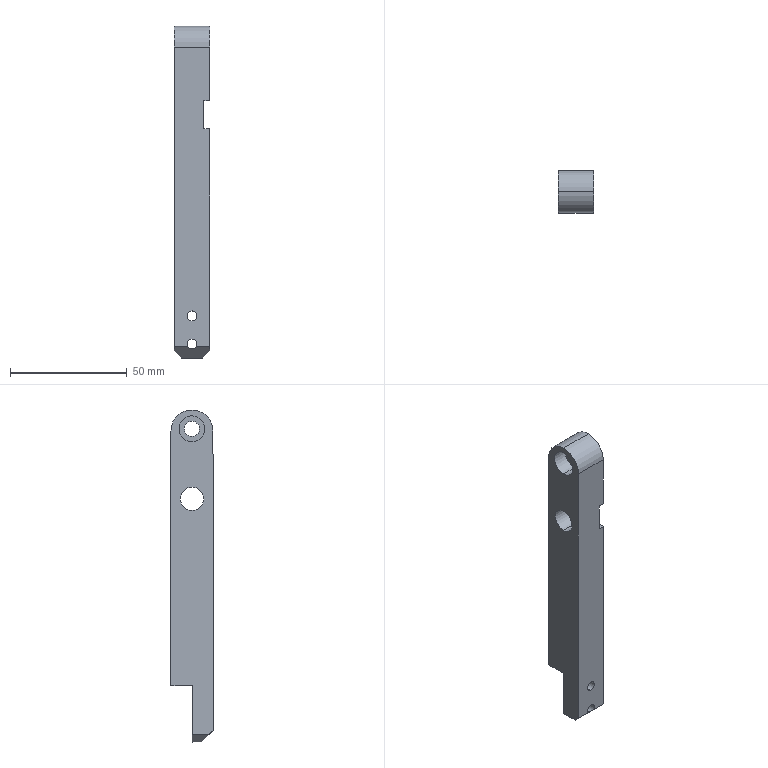Component | SolidWorks | ClampingArm2-1_A87-1 | 1 solid | 30 faces | box 15 x 18.04 x 142 mm | volume 31435 mm3 | plane 16 | cylinder 14 | commonest cylinder face diameters 4.2 x4 11 x2 14 x2 10 x2 6.5 x2 18 x2 | material S45C
STEP:
#1=COLOUR_RGB('',0.7922,0.8196,0.9333);
#2=FILL_AREA_STYLE_COLOUR('',#1);
#3=FILL_AREA_STYLE('',(#2));
#4=SURFACE_STYLE_FILL_AREA(#3);
#5=SURFACE_SIDE_STYLE('',(#4));
#6=SURFACE_STYLE_USAGE(.BOTH.,#5);
#7=PRESENTATION_STYLE_ASSIGNMENT((#6));
#8=CARTESIAN_POINT('',(-1.768,2.244,-5.964));
#9=VERTEX_POINT('',#8);
#10=CARTESIAN_POINT('',(-1.695,2.287,-6.008));
#11=VERTEX_POINT('',#10);
#12=CARTESIAN_POINT('',(-1.768,2.244,-5.964));
#13=CARTESIAN_POINT('',(-1.753,2.272,-5.992));
#14=CARTESIAN_POINT('',(-1.726,2.287,-6.008));
#15=CARTESIAN_POINT('',(-1.695,2.287,-6.008));
#16=(BOUNDED_CURVE()B_SPLINE_CURVE(3,(#12,#13,#14,#15),.UNSPECIFIED.,.F.,.F.)B_SPLINE_CURVE_WITH_KNOTS((4,4),(5.209,6.283),.UNSPECIFIED.)CURVE()GEOMETRIC_REPRESENTATION_ITEM()RATIONAL_B_SPLINE_CURVE((1.,0.9061,0.9061,1.))REPRESENTATION_ITEM(''));
#17=EDGE_CURVE('',#9,#11,#16,.T.);
#18=ORIENTED_EDGE('',*,*,#17,.T.);
#19=CARTESIAN_POINT('',(-1.695,2.599,-6.008));
#20=VERTEX_POINT('',#19);
#21=CARTESIAN_POINT('',(-1.695,2.599,-6.008));
#22=DIRECTION('',(-0.,1.,-0.0003333));
#23=VECTOR('',#22,39.37);
#24=LINE('',#21,#23);
#25=EDGE_CURVE('',#11,#20,#24,.T.);
#26=ORIENTED_EDGE('',*,*,#25,.T.);
#27=CARTESIAN_POINT('',(-1.695,2.599,-5.843));
#28=VERTEX_POINT('',#27);
#29=CARTESIAN_POINT('',(-1.695,2.599,-5.925));
#30=DIRECTION('',(-0.,1.,-0.0003333));
#31=DIRECTION('',(0.,0.0003333,1.));
#32=AXIS2_PLACEMENT_3D('',#29,#30,#31);
#33=CIRCLE('',#32,0.08268);
#34=EDGE_CURVE('',#20,#28,#33,.T.);
#35=ORIENTED_EDGE('',*,*,#34,.T.);
#36=CARTESIAN_POINT('',(-1.695,2.244,-5.842));
#37=VERTEX_POINT('',#36);
#38=CARTESIAN_POINT('',(-1.695,2.599,-5.843));
#39=DIRECTION('',(-0.,1.,-0.0003333));
#40=VECTOR('',#39,39.37);
#41=LINE('',#38,#40);
#42=EDGE_CURVE('',#37,#28,#41,.T.);
#43=ORIENTED_EDGE('',*,*,#42,.F.);
#44=CARTESIAN_POINT('',(-1.695,2.244,-5.925));
#45=DIRECTION('',(-0.,1.,-0.0003333));
#46=DIRECTION('',(0.,0.0003333,1.));
#47=AXIS2_PLACEMENT_3D('',#44,#45,#46);
#48=CIRCLE('',#47,0.08268);
#49=EDGE_CURVE('',#9,#37,#48,.T.);
#50=ORIENTED_EDGE('',*,*,#49,.F.);
#51=EDGE_LOOP('',(#18,#26,#35,#43,#50));
#52=FACE_OUTER_BOUND('',#51,.T.);
#53=CARTESIAN_POINT('',(-1.695,2.599,-5.925));
#54=DIRECTION('',(-0.,1.,-0.0003333));
#55=DIRECTION('',(0.,0.0003333,1.));
#56=AXIS2_PLACEMENT_3D('',#53,#54,#55);
#57=CYLINDRICAL_SURFACE('',#56,0.08268);
#58=ADVANCED_FACE('',(#52),#57,.F.);
#59=CARTESIAN_POINT('',(-1.695,2.244,-5.535));
#60=VERTEX_POINT('',#59);
#61=CARTESIAN_POINT('',(-1.695,2.244,-5.37));
#62=VERTEX_POINT('',#61);
#63=CARTESIAN_POINT('',(-1.695,2.244,-5.453));
#64=DIRECTION('',(-0.,1.,-0.0003333));
#65=DIRECTION('',(0.,0.0003333,1.));
#66=AXIS2_PLACEMENT_3D('',#63,#64,#65);
#67=CIRCLE('',#66,0.08268);
#68=EDGE_CURVE('',#60,#62,#67,.T.);
#69=ORIENTED_EDGE('',*,*,#68,.F.);
#70=CARTESIAN_POINT('',(-1.695,2.599,-5.535));
#71=VERTEX_POINT('',#70);
#72=CARTESIAN_POINT('',(-1.695,2.599,-5.535));
#73=DIRECTION('',(-0.,1.,-0.0003333));
#74=VECTOR('',#73,39.37);
#75=LINE('',#72,#74);
#76=EDGE_CURVE('',#60,#71,#75,.T.);
#77=ORIENTED_EDGE('',*,*,#76,.T.);
#78=CARTESIAN_POINT('',(-1.695,2.599,-5.37));
#79=VERTEX_POINT('',#78);
#80=CARTESIAN_POINT('',(-1.695,2.599,-5.453));
#81=DIRECTION('',(-0.,1.,-0.0003333));
#82=DIRECTION('',(0.,0.0003333,1.));
#83=AXIS2_PLACEMENT_3D('',#80,#81,#82);
#84=CIRCLE('',#83,0.08268);
#85=EDGE_CURVE('',#71,#79,#84,.T.);
#86=ORIENTED_EDGE('',*,*,#85,.T.);
#87=CARTESIAN_POINT('',(-1.695,2.599,-5.37));
#88=DIRECTION('',(-0.,1.,-0.0003333));
#89=VECTOR('',#88,39.37);
#90=LINE('',#87,#89);
#91=EDGE_CURVE('',#62,#79,#90,.T.);
#92=ORIENTED_EDGE('',*,*,#91,.F.);
#93=EDGE_LOOP('',(#69,#77,#86,#92));
#94=FACE_OUTER_BOUND('',#93,.T.);
#95=CARTESIAN_POINT('',(-1.695,2.599,-5.453));
#96=DIRECTION('',(-0.,1.,-0.0003333));
#97=DIRECTION('',(0.,0.0003333,1.));
#98=AXIS2_PLACEMENT_3D('',#95,#96,#97);
#99=CYLINDRICAL_SURFACE('',#98,0.08268);
#100=ADVANCED_FACE('',(#94),#99,.F.);
#101=CARTESIAN_POINT('',(-1.734,2.6,-1.102));
#102=VERTEX_POINT('',#101);
#103=CARTESIAN_POINT('',(-1.734,2.6,-0.6693));
#104=VERTEX_POINT('',#103);
#105=CARTESIAN_POINT('',(-1.734,2.6,-0.8858));
#106=DIRECTION('',(-1.,-0.,0.));
#107=DIRECTION('',(0.,0.0003333,1.));
#108=AXIS2_PLACEMENT_3D('',#105,#106,#107);
#109=CIRCLE('',#108,0.2165);
#110=EDGE_CURVE('',#102,#104,#109,.T.);
#111=ORIENTED_EDGE('',*,*,#110,.F.);
#112=CARTESIAN_POINT('',(-1.99,2.6,-1.102));
#113=VERTEX_POINT('',#112);
#114=CARTESIAN_POINT('',(-1.734,2.6,-1.102));
#115=DIRECTION('',(-1.,-0.,0.));
#116=VECTOR('',#115,39.37);
#117=LINE('',#114,#116);
#118=EDGE_CURVE('',#102,#113,#117,.T.);
#119=ORIENTED_EDGE('',*,*,#118,.T.);
#120=CARTESIAN_POINT('',(-1.99,2.6,-0.6693));
#121=VERTEX_POINT('',#120);
#122=CARTESIAN_POINT('',(-1.99,2.6,-0.8858));
#123=DIRECTION('',(-1.,-0.,0.));
#124=DIRECTION('',(0.,0.0003333,1.));
#125=AXIS2_PLACEMENT_3D('',#122,#123,#124);
#126=CIRCLE('',#125,0.2165);
#127=EDGE_CURVE('',#113,#121,#126,.T.);
#128=ORIENTED_EDGE('',*,*,#127,.T.);
#129=CARTESIAN_POINT('',(-1.734,2.6,-0.6693));
#130=DIRECTION('',(-1.,-0.,0.));
#131=VECTOR('',#130,39.37);
#132=LINE('',#129,#131);
#133=EDGE_CURVE('',#104,#121,#132,.T.);
#134=ORIENTED_EDGE('',*,*,#133,.F.);
#135=EDGE_LOOP('',(#111,#119,#128,#134));
#136=FACE_OUTER_BOUND('',#135,.T.);
#137=CARTESIAN_POINT('',(-1.734,2.6,-0.8858));
#138=DIRECTION('',(-1.,-0.,0.));
#139=DIRECTION('',(0.,0.0003333,1.));
#140=AXIS2_PLACEMENT_3D('',#137,#138,#139);
#141=CYLINDRICAL_SURFACE('',#140,0.2165);
#142=ADVANCED_FACE('',(#136),#141,.F.);
#143=CARTESIAN_POINT('',(-1.478,2.6,-0.6102));
#144=VERTEX_POINT('',#143);
#145=CARTESIAN_POINT('',(-1.478,2.6,-1.161));
#146=VERTEX_POINT('',#145);
#147=CARTESIAN_POINT('',(-1.478,2.6,-0.8858));
#148=DIRECTION('',(1.,0.,-0.));
#149=DIRECTION('',(0.,-0.0003333,-1.));
#150=AXIS2_PLACEMENT_3D('',#147,#148,#149);
#151=CIRCLE('',#150,0.2756);
#152=EDGE_CURVE('',#144,#146,#151,.T.);
#153=ORIENTED_EDGE('',*,*,#152,.F.);
#154=CARTESIAN_POINT('',(-1.4,2.6,-0.6102));
#155=VERTEX_POINT('',#154);
#156=CARTESIAN_POINT('',(-1.478,2.6,-0.6102));
#157=DIRECTION('',(1.,0.,-0.));
#158=VECTOR('',#157,39.37);
#159=LINE('',#156,#158);
#160=EDGE_CURVE('',#144,#155,#159,.T.);
#161=ORIENTED_EDGE('',*,*,#160,.T.);
#162=CARTESIAN_POINT('',(-1.4,2.6,-1.161));
#163=VERTEX_POINT('',#162);
#164=CARTESIAN_POINT('',(-1.4,2.6,-0.8858));
#165=DIRECTION('',(1.,0.,-0.));
#166=DIRECTION('',(0.,-0.0003333,-1.));
#167=AXIS2_PLACEMENT_3D('',#164,#165,#166);
#168=CIRCLE('',#167,0.2756);
#169=EDGE_CURVE('',#155,#163,#168,.T.);
#170=ORIENTED_EDGE('',*,*,#169,.T.);
#171=CARTESIAN_POINT('',(-1.478,2.6,-1.161));
#172=DIRECTION('',(1.,0.,-0.));
#173=VECTOR('',#172,39.37);
#174=LINE('',#171,#173);
#175=EDGE_CURVE('',#146,#163,#174,.T.);
#176=ORIENTED_EDGE('',*,*,#175,.F.);
#177=EDGE_LOOP('',(#153,#161,#170,#176));
#178=FACE_OUTER_BOUND('',#177,.T.);
#179=CARTESIAN_POINT('',(-1.478,2.6,-0.8858));
#180=DIRECTION('',(1.,0.,-0.));
#181=DIRECTION('',(0.,-0.0003333,-1.));
#182=AXIS2_PLACEMENT_3D('',#179,#180,#181);
#183=CYLINDRICAL_SURFACE('',#182,0.2756);
#184=ADVANCED_FACE('',(#178),#183,.F.);
#185=CARTESIAN_POINT('',(-1.99,2.6,-1.87));
#186=VERTEX_POINT('',#185);
#187=CARTESIAN_POINT('',(-1.99,2.6,-2.264));
#188=VERTEX_POINT('',#187);
#189=CARTESIAN_POINT('',(-1.99,2.6,-2.067));
#190=DIRECTION('',(1.,0.,-0.));
#191=DIRECTION('',(0.,-0.0003333,-1.));
#192=AXIS2_PLACEMENT_3D('',#189,#190,#191);
#193=CIRCLE('',#192,0.1969);
#194=EDGE_CURVE('',#186,#188,#193,.T.);
#195=ORIENTED_EDGE('',*,*,#194,.F.);
#196=CARTESIAN_POINT('',(-1.498,2.6,-1.87));
#197=VERTEX_POINT('',#196);
#198=CARTESIAN_POINT('',(-1.99,2.6,-1.87));
#199=DIRECTION('',(1.,0.,-0.));
#200=VECTOR('',#199,39.37);
#201=LINE('',#198,#200);
#202=EDGE_CURVE('',#186,#197,#201,.T.);
#203=ORIENTED_EDGE('',*,*,#202,.T.);
#204=CARTESIAN_POINT('',(-1.498,2.6,-2.264));
#205=VERTEX_POINT('',#204);
#206=CARTESIAN_POINT('',(-1.498,2.6,-2.067));
#207=DIRECTION('',(1.,0.,-0.));
#208=DIRECTION('',(0.,0.0003333,1.));
#209=AXIS2_PLACEMENT_3D('',#206,#207,#208);
#210=CIRCLE('',#209,0.1969);
#211=EDGE_CURVE('',#197,#205,#210,.T.);
#212=ORIENTED_EDGE('',*,*,#211,.T.);
#213=CARTESIAN_POINT('',(-1.99,2.6,-2.264));
#214=DIRECTION('',(1.,0.,-0.));
#215=VECTOR('',#214,39.37);
#216=LINE('',#213,#215);
#217=EDGE_CURVE('',#188,#205,#216,.T.);
#218=ORIENTED_EDGE('',*,*,#217,.F.);
#219=EDGE_LOOP('',(#195,#203,#212,#218));
#220=FACE_OUTER_BOUND('',#219,.T.);
#221=CARTESIAN_POINT('',(-1.99,2.6,-2.067));
#222=DIRECTION('',(1.,0.,-0.));
#223=DIRECTION('',(0.,-0.0003333,-1.));
#224=AXIS2_PLACEMENT_3D('',#221,#222,#223);
#225=CYLINDRICAL_SURFACE('',#224,0.1969);
#226=ADVANCED_FACE('',(#220),#225,.F.);
#227=CARTESIAN_POINT('',(-1.734,2.6,-0.7579));
#228=VERTEX_POINT('',#227);
#229=CARTESIAN_POINT('',(-1.734,2.6,-1.014));
#230=VERTEX_POINT('',#229);
#231=CARTESIAN_POINT('',(-1.734,2.6,-0.8858));
#232=DIRECTION('',(1.,0.,-0.));
#233=DIRECTION('',(0.,0.0003333,1.));
#234=AXIS2_PLACEMENT_3D('',#231,#232,#233);
#235=CIRCLE('',#234,0.128);
#236=EDGE_CURVE('',#228,#230,#235,.T.);
#237=ORIENTED_EDGE('',*,*,#236,.F.);
#238=CARTESIAN_POINT('',(-1.478,2.6,-0.7579));
#239=VERTEX_POINT('',#238);
#240=CARTESIAN_POINT('',(-1.99,2.6,-0.7579));
#241=DIRECTION('',(1.,0.,-0.));
#242=VECTOR('',#241,39.37);
#243=LINE('',#240,#242);
#244=EDGE_CURVE('',#228,#239,#243,.T.);
#245=ORIENTED_EDGE('',*,*,#244,.T.);
#246=CARTESIAN_POINT('',(-1.478,2.6,-1.014));
#247=VERTEX_POINT('',#246);
#248=CARTESIAN_POINT('',(-1.478,2.6,-0.8858));
#249=DIRECTION('',(-1.,-0.,0.));
#250=DIRECTION('',(0.,-0.0003333,-1.));
#251=AXIS2_PLACEMENT_3D('',#248,#249,#250);
#252=CIRCLE('',#251,0.128);
#253=EDGE_CURVE('',#247,#239,#252,.T.);
#254=ORIENTED_EDGE('',*,*,#253,.F.);
#255=CARTESIAN_POINT('',(-1.99,2.6,-1.014));
#256=DIRECTION('',(1.,0.,-0.));
#257=VECTOR('',#256,39.37);
#258=LINE('',#255,#257);
#259=EDGE_CURVE('',#230,#247,#258,.T.);
#260=ORIENTED_EDGE('',*,*,#259,.F.);
#261=EDGE_LOOP('',(#237,#245,#254,#260));
#262=FACE_OUTER_BOUND('',#261,.T.);
#263=CARTESIAN_POINT('',(-1.99,2.6,-0.8858));
#264=DIRECTION('',(1.,0.,-0.));
#265=DIRECTION('',(0.,-0.0003333,-1.));
#266=AXIS2_PLACEMENT_3D('',#263,#264,#265);
#267=CYLINDRICAL_SURFACE('',#266,0.128);
#268=ADVANCED_FACE('',(#262),#267,.F.);
#269=ORIENTED_EDGE('',*,*,#244,.F.);
#270=CARTESIAN_POINT('',(-1.734,2.6,-0.8858));
#271=DIRECTION('',(1.,0.,-0.));
#272=DIRECTION('',(0.,0.0003333,1.));
#273=AXIS2_PLACEMENT_3D('',#270,#271,#272);
#274=CIRCLE('',#273,0.128);
#275=EDGE_CURVE('',#230,#228,#274,.T.);
#276=ORIENTED_EDGE('',*,*,#275,.F.);
#277=ORIENTED_EDGE('',*,*,#259,.T.);
#278=CARTESIAN_POINT('',(-1.478,2.6,-0.8858));
#279=DIRECTION('',(-1.,-0.,0.));
#280=DIRECTION('',(0.,-0.0003333,-1.));
#281=AXIS2_PLACEMENT_3D('',#278,#279,#280);
#282=CIRCLE('',#281,0.128);
#283=EDGE_CURVE('',#239,#247,#282,.T.);
#284=ORIENTED_EDGE('',*,*,#283,.F.);
#285=EDGE_LOOP('',(#269,#276,#277,#284));
#286=FACE_OUTER_BOUND('',#285,.T.);
#287=CARTESIAN_POINT('',(-1.99,2.6,-0.8858));
#288=DIRECTION('',(1.,0.,-0.));
#289=DIRECTION('',(0.,-0.0003333,-1.));
#290=AXIS2_PLACEMENT_3D('',#287,#288,#289);
#291=CYLINDRICAL_SURFACE('',#290,0.128);
#292=ADVANCED_FACE('',(#286),#291,.F.);
#293=CARTESIAN_POINT('',(-1.4,2.6,-0.8858));
#294=DIRECTION('',(1.,0.,-0.));
#295=DIRECTION('',(0.,-0.0003333,-1.));
#296=AXIS2_PLACEMENT_3D('',#293,#294,#295);
#297=CIRCLE('',#296,0.2756);
#298=EDGE_CURVE('',#163,#155,#297,.T.);
#299=ORIENTED_EDGE('',*,*,#298,.F.);
#300=ORIENTED_EDGE('',*,*,#169,.F.);
#301=EDGE_LOOP('',(#299,#300));
#302=FACE_BOUND('',#301,.T.);
#303=CARTESIAN_POINT('',(-1.4,2.954,-1.831));
#304=VERTEX_POINT('',#303);
#305=CARTESIAN_POINT('',(-1.4,2.955,-0.9253));
#306=VERTEX_POINT('',#305);
#307=CARTESIAN_POINT('',(-1.4,2.955,-0.571));
#308=DIRECTION('',(0.,0.0003333,1.));
#309=VECTOR('',#308,39.37);
#310=LINE('',#307,#309);
#311=EDGE_CURVE('',#304,#306,#310,.T.);
#312=ORIENTED_EDGE('',*,*,#311,.T.);
#313=CARTESIAN_POINT('',(-1.4,2.6,-0.5709));
#314=VERTEX_POINT('',#313);
#315=CARTESIAN_POINT('',(-1.4,2.6,-0.9252));
#316=DIRECTION('',(1.,0.,-0.));
#317=DIRECTION('',(0.,-0.0003333,-1.));
#318=AXIS2_PLACEMENT_3D('',#315,#316,#317);
#319=CIRCLE('',#318,0.3543);
#320=EDGE_CURVE('',#306,#314,#319,.T.);
#321=ORIENTED_EDGE('',*,*,#320,.T.);
#322=CARTESIAN_POINT('',(-1.4,2.246,-0.9251));
#323=VERTEX_POINT('',#322);
#324=CARTESIAN_POINT('',(-1.4,2.6,-0.9252));
#325=DIRECTION('',(1.,0.,-0.));
#326=DIRECTION('',(0.,-0.0003333,-1.));
#327=AXIS2_PLACEMENT_3D('',#324,#325,#326);
#328=CIRCLE('',#327,0.3543);
#329=EDGE_CURVE('',#314,#323,#328,.T.);
#330=ORIENTED_EDGE('',*,*,#329,.T.);
#331=CARTESIAN_POINT('',(-1.4,2.246,-1.831));
#332=VERTEX_POINT('',#331);
#333=CARTESIAN_POINT('',(-1.4,2.246,-0.5707));
#334=DIRECTION('',(-0.,-0.0003333,-1.));
#335=VECTOR('',#334,39.37);
#336=LINE('',#333,#335);
#337=EDGE_CURVE('',#323,#332,#336,.T.);
#338=ORIENTED_EDGE('',*,*,#337,.T.);
#339=CARTESIAN_POINT('',(-1.4,2.954,-1.831));
#340=DIRECTION('',(0.,-1.,0.0003333));
#341=VECTOR('',#340,39.37);
#342=LINE('',#339,#341);
#343=EDGE_CURVE('',#304,#332,#342,.T.);
#344=ORIENTED_EDGE('',*,*,#343,.F.);
#345=EDGE_LOOP('',(#312,#321,#330,#338,#344));
#346=FACE_OUTER_BOUND('',#345,.T.);
#347=CARTESIAN_POINT('',(-1.4,2.599,-3.366));
#348=DIRECTION('',(1.,0.,-0.));
#349=DIRECTION('',(-0.,-0.0003333,-1.));
#350=AXIS2_PLACEMENT_3D('',#347,#348,#349);
#351=PLANE('',#350);
#352=ADVANCED_FACE('',(#302,#346),#351,.T.);
#353=CARTESIAN_POINT('',(-1.518,2.598,-6.161));
#354=VERTEX_POINT('',#353);
#355=CARTESIAN_POINT('',(-1.518,2.441,-6.161));
#356=VERTEX_POINT('',#355);
#357=CARTESIAN_POINT('',(-1.518,2.244,-6.161));
#358=DIRECTION('',(0.,-1.,0.0003333));
#359=VECTOR('',#358,39.37);
#360=LINE('',#357,#359);
#361=EDGE_CURVE('',#354,#356,#360,.T.);
#362=ORIENTED_EDGE('',*,*,#361,.T.);
#363=CARTESIAN_POINT('',(-1.872,2.441,-6.161));
#364=VERTEX_POINT('',#363);
#365=CARTESIAN_POINT('',(-1.4,2.441,-6.161));
#366=DIRECTION('',(-1.,-0.,0.));
#367=VECTOR('',#366,39.37);
#368=LINE('',#365,#367);
#369=EDGE_CURVE('',#356,#364,#368,.T.);
#370=ORIENTED_EDGE('',*,*,#369,.T.);
#371=CARTESIAN_POINT('',(-1.872,2.598,-6.161));
#372=VERTEX_POINT('',#371);
#373=CARTESIAN_POINT('',(-1.872,2.953,-6.162));
#374=DIRECTION('',(-0.,1.,-0.0003333));
#375=VECTOR('',#374,39.37);
#376=LINE('',#373,#375);
#377=EDGE_CURVE('',#364,#372,#376,.T.);
#378=ORIENTED_EDGE('',*,*,#377,.T.);
#379=CARTESIAN_POINT('',(-1.99,2.598,-6.161));
#380=DIRECTION('',(1.,0.,-0.));
#381=VECTOR('',#380,39.37);
#382=LINE('',#379,#381);
#383=EDGE_CURVE('',#372,#354,#382,.T.);
#384=ORIENTED_EDGE('',*,*,#383,.T.);
#385=EDGE_LOOP('',(#362,#370,#378,#384));
#386=FACE_OUTER_BOUND('',#385,.T.);
#387=CARTESIAN_POINT('',(-1.4,2.953,-6.162));
#388=DIRECTION('',(0.,0.0003333,1.));
#389=DIRECTION('',(1.,0.,-0.));
#390=AXIS2_PLACEMENT_3D('',#387,#388,#389);
#391=PLANE('',#390);
#392=ADVANCED_FACE('',(#386),#391,.F.);
#393=CARTESIAN_POINT('',(-1.4,2.953,-5.217));
#394=VERTEX_POINT('',#393);
#395=CARTESIAN_POINT('',(-1.4,2.954,-2.303));
#396=VERTEX_POINT('',#395);
#397=CARTESIAN_POINT('',(-1.4,2.955,-0.571));
#398=DIRECTION('',(0.,0.0003333,1.));
#399=VECTOR('',#398,39.37);
#400=LINE('',#397,#399);
#401=EDGE_CURVE('',#394,#396,#400,.T.);
#402=ORIENTED_EDGE('',*,*,#401,.F.);
#403=CARTESIAN_POINT('',(-1.99,2.953,-5.217));
#404=VERTEX_POINT('',#403);
#405=CARTESIAN_POINT('',(-1.99,2.953,-5.217));
#406=DIRECTION('',(1.,0.,-0.));
#407=VECTOR('',#406,39.37);
#408=LINE('',#405,#407);
#409=EDGE_CURVE('',#404,#394,#408,.T.);
#410=ORIENTED_EDGE('',*,*,#409,.F.);
#411=CARTESIAN_POINT('',(-1.99,2.955,-0.9253));
#412=VERTEX_POINT('',#411);
#413=CARTESIAN_POINT('',(-1.99,2.955,-0.571));
#414=DIRECTION('',(0.,0.0003333,1.));
#415=VECTOR('',#414,39.37);
#416=LINE('',#413,#415);
#417=EDGE_CURVE('',#404,#412,#416,.T.);
#418=ORIENTED_EDGE('',*,*,#417,.T.);
#419=CARTESIAN_POINT('',(-1.4,2.955,-0.9253));
#420=DIRECTION('',(1.,0.,-0.));
#421=VECTOR('',#420,39.37);
#422=LINE('',#419,#421);
#423=EDGE_CURVE('',#412,#306,#422,.T.);
#424=ORIENTED_EDGE('',*,*,#423,.T.);
#425=ORIENTED_EDGE('',*,*,#311,.F.);
#426=CARTESIAN_POINT('',(-1.498,2.954,-1.831));
#427=VERTEX_POINT('',#426);
#428=CARTESIAN_POINT('',(-1.498,2.954,-1.831));
#429=DIRECTION('',(1.,0.,-0.));
#430=VECTOR('',#429,39.37);
#431=LINE('',#428,#430);
#432=EDGE_CURVE('',#427,#304,#431,.T.);
#433=ORIENTED_EDGE('',*,*,#432,.F.);
#434=CARTESIAN_POINT('',(-1.498,2.954,-2.303));
#435=VERTEX_POINT('',#434);
#436=CARTESIAN_POINT('',(-1.498,2.954,-2.303));
#437=DIRECTION('',(0.,0.0003333,1.));
#438=VECTOR('',#437,39.37);
#439=LINE('',#436,#438);
#440=EDGE_CURVE('',#435,#427,#439,.T.);
#441=ORIENTED_EDGE('',*,*,#440,.F.);
#442=CARTESIAN_POINT('',(-1.498,2.954,-2.303));
#443=DIRECTION('',(1.,0.,-0.));
#444=VECTOR('',#443,39.37);
#445=LINE('',#442,#444);
#446=EDGE_CURVE('',#435,#396,#445,.T.);
#447=ORIENTED_EDGE('',*,*,#446,.T.);
#448=EDGE_LOOP('',(#402,#410,#418,#424,#425,#433,#441,#447));
#449=FACE_OUTER_BOUND('',#448,.T.);
#450=CARTESIAN_POINT('',(-1.4,2.955,-0.571));
#451=DIRECTION('',(0.,-1.,0.0003333));
#452=DIRECTION('',(-0.,-0.0003333,-1.));
#453=AXIS2_PLACEMENT_3D('',#450,#451,#452);
#454=PLANE('',#453);
#455=ADVANCED_FACE('',(#449),#454,.F.);
#456=CARTESIAN_POINT('',(-1.695,2.244,-5.453));
#457=DIRECTION('',(-0.,1.,-0.0003333));
#458=DIRECTION('',(0.,0.0003333,1.));
#459=AXIS2_PLACEMENT_3D('',#456,#457,#458);
#460=CIRCLE('',#459,0.08268);
#461=EDGE_CURVE('',#62,#60,#460,.T.);
#462=ORIENTED_EDGE('',*,*,#461,.T.);
#463=ORIENTED_EDGE('',*,*,#68,.T.);
#464=EDGE_LOOP('',(#462,#463));
#465=FACE_BOUND('',#464,.T.);
#466=CARTESIAN_POINT('',(-1.99,2.244,-5.964));
#467=VERTEX_POINT('',#466);
#468=CARTESIAN_POINT('',(-1.4,2.244,-5.964));
#469=DIRECTION('',(1.,0.,-0.));
#470=VECTOR('',#469,39.37);
#471=LINE('',#468,#470);
#472=EDGE_CURVE('',#467,#9,#471,.T.);
#473=ORIENTED_EDGE('',*,*,#472,.T.);
#474=ORIENTED_EDGE('',*,*,#49,.T.);
#475=CARTESIAN_POINT('',(-1.622,2.244,-5.964));
#476=VERTEX_POINT('',#475);
#477=CARTESIAN_POINT('',(-1.695,2.244,-5.925));
#478=DIRECTION('',(-0.,1.,-0.0003333));
#479=DIRECTION('',(0.,0.0003333,1.));
#480=AXIS2_PLACEMENT_3D('',#477,#478,#479);
#481=CIRCLE('',#480,0.08268);
#482=EDGE_CURVE('',#37,#476,#481,.T.);
#483=ORIENTED_EDGE('',*,*,#482,.T.);
#484=CARTESIAN_POINT('',(-1.4,2.244,-5.964));
#485=VERTEX_POINT('',#484);
#486=CARTESIAN_POINT('',(-1.4,2.244,-5.964));
#487=DIRECTION('',(1.,0.,-0.));
#488=VECTOR('',#487,39.37);
#489=LINE('',#486,#488);
#490=EDGE_CURVE('',#476,#485,#489,.T.);
#491=ORIENTED_EDGE('',*,*,#490,.T.);
#492=CARTESIAN_POINT('',(-1.4,2.245,-2.303));
#493=VERTEX_POINT('',#492);
#494=CARTESIAN_POINT('',(-1.4,2.246,-0.5707));
#495=DIRECTION('',(-0.,-0.0003333,-1.));
#496=VECTOR('',#495,39.37);
#497=LINE('',#494,#496);
#498=EDGE_CURVE('',#493,#485,#497,.T.);
#499=ORIENTED_EDGE('',*,*,#498,.F.);
#500=CARTESIAN_POINT('',(-1.498,2.245,-2.303));
#501=VERTEX_POINT('',#500);
#502=CARTESIAN_POINT('',(-1.498,2.245,-2.303));
#503=DIRECTION('',(1.,0.,-0.));
#504=VECTOR('',#503,39.37);
#505=LINE('',#502,#504);
#506=EDGE_CURVE('',#501,#493,#505,.T.);
#507=ORIENTED_EDGE('',*,*,#506,.F.);
#508=CARTESIAN_POINT('',(-1.498,2.246,-1.831));
#509=VERTEX_POINT('',#508);
#510=CARTESIAN_POINT('',(-1.498,2.245,-2.303));
#511=DIRECTION('',(-0.,-0.0003333,-1.));
#512=VECTOR('',#511,39.37);
#513=LINE('',#510,#512);
#514=EDGE_CURVE('',#509,#501,#513,.T.);
#515=ORIENTED_EDGE('',*,*,#514,.F.);
#516=CARTESIAN_POINT('',(-1.498,2.246,-1.831));
#517=DIRECTION('',(1.,0.,-0.));
#518=VECTOR('',#517,39.37);
#519=LINE('',#516,#518);
#520=EDGE_CURVE('',#509,#332,#519,.T.);
#521=ORIENTED_EDGE('',*,*,#520,.T.);
#522=ORIENTED_EDGE('',*,*,#337,.F.);
#523=CARTESIAN_POINT('',(-1.99,2.246,-0.9251));
#524=VERTEX_POINT('',#523);
#525=CARTESIAN_POINT('',(-1.4,2.246,-0.9251));
#526=DIRECTION('',(-1.,-0.,0.));
#527=VECTOR('',#526,39.37);
#528=LINE('',#525,#527);
#529=EDGE_CURVE('',#323,#524,#528,.T.);
#530=ORIENTED_EDGE('',*,*,#529,.T.);
#531=CARTESIAN_POINT('',(-1.99,2.246,-0.5707));
#532=DIRECTION('',(-0.,-0.0003333,-1.));
#533=VECTOR('',#532,39.37);
#534=LINE('',#531,#533);
#535=EDGE_CURVE('',#524,#467,#534,.T.);
#536=ORIENTED_EDGE('',*,*,#535,.T.);
#537=EDGE_LOOP('',(#473,#474,#483,#491,#499,#507,#515,#521,#522,#530,#536));
#538=FACE_OUTER_BOUND('',#537,.T.);
#539=CARTESIAN_POINT('',(-1.4,2.246,-0.5707));
#540=DIRECTION('',(-0.,1.,-0.0003333));
#541=DIRECTION('',(0.,0.0003333,1.));
#542=AXIS2_PLACEMENT_3D('',#539,#540,#541);
#543=PLANE('',#542);
#544=ADVANCED_FACE('',(#465,#538),#543,.F.);
#545=ORIENTED_EDGE('',*,*,#498,.T.);
#546=CARTESIAN_POINT('',(-1.4,2.323,-6.043));
#547=VERTEX_POINT('',#546);
#548=CARTESIAN_POINT('',(-1.4,1.123,-4.842));
#549=DIRECTION('',(-0.,0.7069,-0.7073));
#550=VECTOR('',#549,39.37);
#551=LINE('',#548,#550);
#552=EDGE_CURVE('',#485,#547,#551,.T.);
#553=ORIENTED_EDGE('',*,*,#552,.T.);
#554=CARTESIAN_POINT('',(-1.4,2.599,-6.043));
#555=VERTEX_POINT('',#554);
#556=CARTESIAN_POINT('',(-1.4,2.599,-6.043));
#557=DIRECTION('',(-0.,1.,-0.0003333));
#558=VECTOR('',#557,39.37);
#559=LINE('',#556,#558);
#560=EDGE_CURVE('',#547,#555,#559,.T.);
#561=ORIENTED_EDGE('',*,*,#560,.T.);
#562=CARTESIAN_POINT('',(-1.4,2.599,-5.217));
#563=VERTEX_POINT('',#562);
#564=CARTESIAN_POINT('',(-1.4,2.598,-6.161));
#565=DIRECTION('',(-0.,-0.0003333,-1.));
#566=VECTOR('',#565,39.37);
#567=LINE('',#564,#566);
#568=EDGE_CURVE('',#563,#555,#567,.T.);
#569=ORIENTED_EDGE('',*,*,#568,.F.);
#570=CARTESIAN_POINT('',(-1.4,2.953,-5.217));
#571=DIRECTION('',(0.,-1.,0.0003333));
#572=VECTOR('',#571,39.37);
#573=LINE('',#570,#572);
#574=EDGE_CURVE('',#394,#563,#573,.T.);
#575=ORIENTED_EDGE('',*,*,#574,.F.);
#576=ORIENTED_EDGE('',*,*,#401,.T.);
#577=CARTESIAN_POINT('',(-1.4,2.954,-2.303));
#578=DIRECTION('',(-0.,1.,-0.0003333));
#579=VECTOR('',#578,39.37);
#580=LINE('',#577,#579);
#581=EDGE_CURVE('',#493,#396,#580,.T.);
#582=ORIENTED_EDGE('',*,*,#581,.F.);
#583=EDGE_LOOP('',(#545,#553,#561,#569,#575,#576,#582));
#584=FACE_OUTER_BOUND('',#583,.T.);
#585=CARTESIAN_POINT('',(-1.4,2.599,-3.366));
#586=DIRECTION('',(1.,0.,-0.));
#587=DIRECTION('',(-0.,-0.0003333,-1.));
#588=AXIS2_PLACEMENT_3D('',#585,#586,#587);
#589=PLANE('',#588);
#590=ADVANCED_FACE('',(#584),#589,.T.);
#591=CARTESIAN_POINT('',(-1.99,2.6,-0.8858));
#592=DIRECTION('',(-1.,-0.,0.));
#593=DIRECTION('',(0.,0.0003333,1.));
#594=AXIS2_PLACEMENT_3D('',#591,#592,#593);
#595=CIRCLE('',#594,0.2165);
#596=EDGE_CURVE('',#121,#113,#595,.T.);
#597=ORIENTED_EDGE('',*,*,#596,.F.);
#598=ORIENTED_EDGE('',*,*,#127,.F.);
#599=EDGE_LOOP('',(#597,#598));
#600=FACE_BOUND('',#599,.T.);
#601=CARTESIAN_POINT('',(-1.99,2.6,-2.067));
#602=DIRECTION('',(1.,0.,-0.));
#603=DIRECTION('',(0.,-0.0003333,-1.));
#604=AXIS2_PLACEMENT_3D('',#601,#602,#603);
#605=CIRCLE('',#604,0.1969);
#606=EDGE_CURVE('',#188,#186,#605,.T.);
#607=ORIENTED_EDGE('',*,*,#606,.T.);
#608=ORIENTED_EDGE('',*,*,#194,.T.);
#609=EDGE_LOOP('',(#607,#608));
#610=FACE_BOUND('',#609,.T.);
#611=CARTESIAN_POINT('',(-1.99,2.599,-6.043));
#612=VERTEX_POINT('',#611);
#613=CARTESIAN_POINT('',(-1.99,2.323,-6.043));
#614=VERTEX_POINT('',#613);
#615=CARTESIAN_POINT('',(-1.99,2.599,-6.043));
#616=DIRECTION('',(0.,-1.,0.0003333));
#617=VECTOR('',#616,39.37);
#618=LINE('',#615,#617);
#619=EDGE_CURVE('',#612,#614,#618,.T.);
#620=ORIENTED_EDGE('',*,*,#619,.T.);
#621=CARTESIAN_POINT('',(-1.99,2.441,-6.161));
#622=DIRECTION('',(0.,-0.7069,0.7073));
#623=VECTOR('',#622,39.37);
#624=LINE('',#621,#623);
#625=EDGE_CURVE('',#614,#467,#624,.T.);
#626=ORIENTED_EDGE('',*,*,#625,.T.);
#627=ORIENTED_EDGE('',*,*,#535,.F.);
#628=CARTESIAN_POINT('',(-1.99,2.6,-0.5709));
#629=VERTEX_POINT('',#628);
#630=CARTESIAN_POINT('',(-1.99,2.6,-0.9252));
#631=DIRECTION('',(-1.,-0.,0.));
#632=DIRECTION('',(0.,-0.0003333,-1.));
#633=AXIS2_PLACEMENT_3D('',#630,#631,#632);
#634=CIRCLE('',#633,0.3543);
#635=EDGE_CURVE('',#524,#629,#634,.T.);
#636=ORIENTED_EDGE('',*,*,#635,.T.);
#637=CARTESIAN_POINT('',(-1.99,2.6,-0.9252));
#638=DIRECTION('',(-1.,-0.,0.));
#639=DIRECTION('',(0.,-0.0003333,-1.));
#640=AXIS2_PLACEMENT_3D('',#637,#638,#639);
#641=CIRCLE('',#640,0.3543);
#642=EDGE_CURVE('',#629,#412,#641,.T.);
#643=ORIENTED_EDGE('',*,*,#642,.T.);
#644=ORIENTED_EDGE('',*,*,#417,.F.);
#645=CARTESIAN_POINT('',(-1.99,2.599,-5.217));
#646=VERTEX_POINT('',#645);
#647=CARTESIAN_POINT('',(-1.99,2.953,-5.217));
#648=DIRECTION('',(0.,-1.,0.0003333));
#649=VECTOR('',#648,39.37);
#650=LINE('',#647,#649);
#651=EDGE_CURVE('',#404,#646,#650,.T.);
#652=ORIENTED_EDGE('',*,*,#651,.T.);
#653=CARTESIAN_POINT('',(-1.99,2.598,-6.161));
#654=DIRECTION('',(-0.,-0.0003333,-1.));
#655=VECTOR('',#654,39.37);
#656=LINE('',#653,#655);
#657=EDGE_CURVE('',#646,#612,#656,.T.);
#658=ORIENTED_EDGE('',*,*,#657,.T.);
#659=EDGE_LOOP('',(#620,#626,#627,#636,#643,#644,#652,#658));
#660=FACE_OUTER_BOUND('',#659,.T.);
#661=CARTESIAN_POINT('',(-1.99,2.599,-3.366));
#662=DIRECTION('',(1.,0.,-0.));
#663=DIRECTION('',(-0.,-0.0003333,-1.));
#664=AXIS2_PLACEMENT_3D('',#661,#662,#663);
#665=PLANE('',#664);
#666=ADVANCED_FACE('',(#600,#610,#660),#665,.F.);
#667=ORIENTED_EDGE('',*,*,#202,.F.);
#668=ORIENTED_EDGE('',*,*,#606,.F.);
#669=ORIENTED_EDGE('',*,*,#217,.T.);
#670=CARTESIAN_POINT('',(-1.498,2.6,-2.067));
#671=DIRECTION('',(1.,0.,-0.));
#672=DIRECTION('',(0.,0.0003333,1.));
#673=AXIS2_PLACEMENT_3D('',#670,#671,#672);
#674=CIRCLE('',#673,0.1969);
#675=EDGE_CURVE('',#205,#197,#674,.T.);
#676=ORIENTED_EDGE('',*,*,#675,.T.);
#677=EDGE_LOOP('',(#667,#668,#669,#676));
#678=FACE_OUTER_BOUND('',#677,.T.);
#679=CARTESIAN_POINT('',(-1.99,2.6,-2.067));
#680=DIRECTION('',(1.,0.,-0.));
#681=DIRECTION('',(0.,-0.0003333,-1.));
#682=AXIS2_PLACEMENT_3D('',#679,#680,#681);
#683=CYLINDRICAL_SURFACE('',#682,0.1969);
#684=ADVANCED_FACE('',(#678),#683,.F.);
#685=CARTESIAN_POINT('',(-1.498,2.954,-1.831));
#686=DIRECTION('',(0.,-1.,0.0003333));
#687=VECTOR('',#686,39.37);
#688=LINE('',#685,#687);
#689=EDGE_CURVE('',#427,#509,#688,.T.);
#690=ORIENTED_EDGE('',*,*,#689,.T.);
#691=ORIENTED_EDGE('',*,*,#514,.T.);
#692=CARTESIAN_POINT('',(-1.498,2.954,-2.303));
#693=DIRECTION('',(-0.,1.,-0.0003333));
#694=VECTOR('',#693,39.37);
#695=LINE('',#692,#694);
#696=EDGE_CURVE('',#501,#435,#695,.T.);
#697=ORIENTED_EDGE('',*,*,#696,.T.);
#698=ORIENTED_EDGE('',*,*,#440,.T.);
#699=EDGE_LOOP('',(#690,#691,#697,#698));
#700=FACE_OUTER_BOUND('',#699,.T.);
#701=ORIENTED_EDGE('',*,*,#675,.F.);
#702=ORIENTED_EDGE('',*,*,#211,.F.);
#703=EDGE_LOOP('',(#701,#702));
#704=FACE_BOUND('',#703,.T.);
#705=CARTESIAN_POINT('',(-1.498,2.599,-3.366));
#706=DIRECTION('',(-1.,-0.,0.));
#707=DIRECTION('',(0.,0.0003333,1.));
#708=AXIS2_PLACEMENT_3D('',#705,#706,#707);
#709=PLANE('',#708);
#710=ADVANCED_FACE('',(#700,#704),#709,.F.);
#711=ORIENTED_EDGE('',*,*,#343,.T.);
#712=ORIENTED_EDGE('',*,*,#520,.F.);
#713=ORIENTED_EDGE('',*,*,#689,.F.);
#714=ORIENTED_EDGE('',*,*,#432,.T.);
#715=EDGE_LOOP('',(#711,#712,#713,#714));
#716=FACE_OUTER_BOUND('',#715,.T.);
#717=CARTESIAN_POINT('',(-1.498,2.954,-1.831));
#718=DIRECTION('',(0.,0.0003333,1.));
#719=DIRECTION('',(1.,0.,-0.));
#720=AXIS2_PLACEMENT_3D('',#717,#718,#719);
#721=PLANE('',#720);
#722=ADVANCED_FACE('',(#716),#721,.F.);
#723=ORIENTED_EDGE('',*,*,#581,.T.);
#724=ORIENTED_EDGE('',*,*,#446,.F.);
#725=ORIENTED_EDGE('',*,*,#696,.F.);
#726=ORIENTED_EDGE('',*,*,#506,.T.);
#727=EDGE_LOOP('',(#723,#724,#725,#726));
#728=FACE_OUTER_BOUND('',#727,.T.);
#729=CARTESIAN_POINT('',(-1.498,2.954,-2.303));
#730=DIRECTION('',(-0.,-0.0003333,-1.));
#731=DIRECTION('',(-1.,-0.,0.));
#732=AXIS2_PLACEMENT_3D('',#729,#730,#731);
#733=PLANE('',#732);
#734=ADVANCED_FACE('',(#728),#733,.F.);
#735=ORIENTED_EDGE('',*,*,#529,.F.);
#736=ORIENTED_EDGE('',*,*,#329,.F.);
#737=CARTESIAN_POINT('',(-1.4,2.6,-0.5709));
#738=DIRECTION('',(1.,0.,-0.));
#739=VECTOR('',#738,39.37);
#740=LINE('',#737,#739);
#741=EDGE_CURVE('',#629,#314,#740,.T.);
#742=ORIENTED_EDGE('',*,*,#741,.F.);
#743=ORIENTED_EDGE('',*,*,#635,.F.);
#744=EDGE_LOOP('',(#735,#736,#742,#743));
#745=FACE_OUTER_BOUND('',#744,.T.);
#746=CARTESIAN_POINT('',(-1.4,2.6,-0.9252));
#747=DIRECTION('',(-1.,-0.,0.));
#748=DIRECTION('',(0.,0.0003333,1.));
#749=AXIS2_PLACEMENT_3D('',#746,#747,#748);
#750=CYLINDRICAL_SURFACE('',#749,0.3543);
#751=ADVANCED_FACE('',(#745),#750,.T.);
#752=ORIENTED_EDGE('',*,*,#320,.F.);
#753=ORIENTED_EDGE('',*,*,#423,.F.);
#754=ORIENTED_EDGE('',*,*,#642,.F.);
#755=ORIENTED_EDGE('',*,*,#741,.T.);
#756=EDGE_LOOP('',(#752,#753,#754,#755));
#757=FACE_OUTER_BOUND('',#756,.T.);
#758=CARTESIAN_POINT('',(-1.4,2.6,-0.9252));
#759=DIRECTION('',(-1.,-0.,0.));
#760=DIRECTION('',(0.,0.0003333,1.));
#761=AXIS2_PLACEMENT_3D('',#758,#759,#760);
#762=CYLINDRICAL_SURFACE('',#761,0.3543);
#763=ADVANCED_FACE('',(#757),#762,.T.);
#764=CARTESIAN_POINT('',(-1.478,2.6,-0.8858));
#765=DIRECTION('',(1.,0.,-0.));
#766=DIRECTION('',(0.,-0.0003333,-1.));
#767=AXIS2_PLACEMENT_3D('',#764,#765,#766);
#768=CIRCLE('',#767,0.2756);
#769=EDGE_CURVE('',#146,#144,#768,.T.);
#770=ORIENTED_EDGE('',*,*,#769,.T.);
#771=ORIENTED_EDGE('',*,*,#152,.T.);
#772=EDGE_LOOP('',(#770,#771));
#773=FACE_OUTER_BOUND('',#772,.T.);
#774=ORIENTED_EDGE('',*,*,#253,.T.);
#775=ORIENTED_EDGE('',*,*,#283,.T.);
#776=EDGE_LOOP('',(#774,#775));
#777=FACE_BOUND('',#776,.T.);
#778=CARTESIAN_POINT('',(-1.478,2.6,-0.8858));
#779=DIRECTION('',(1.,0.,-0.));
#780=DIRECTION('',(-0.,-0.0003333,-1.));
#781=AXIS2_PLACEMENT_3D('',#778,#779,#780);
#782=PLANE('',#781);
#783=ADVANCED_FACE('',(#773,#777),#782,.T.);
#784=ORIENTED_EDGE('',*,*,#160,.F.);
#785=ORIENTED_EDGE('',*,*,#769,.F.);
#786=ORIENTED_EDGE('',*,*,#175,.T.);
#787=ORIENTED_EDGE('',*,*,#298,.T.);
#788=EDGE_LOOP('',(#784,#785,#786,#787));
#789=FACE_OUTER_BOUND('',#788,.T.);
#790=CARTESIAN_POINT('',(-1.478,2.6,-0.8858));
#791=DIRECTION('',(1.,0.,-0.));
#792=DIRECTION('',(0.,-0.0003333,-1.));
#793=AXIS2_PLACEMENT_3D('',#790,#791,#792);
#794=CYLINDRICAL_SURFACE('',#793,0.2756);
#795=ADVANCED_FACE('',(#789),#794,.F.);
#796=CARTESIAN_POINT('',(-1.734,2.6,-0.8858));
#797=DIRECTION('',(-1.,-0.,0.));
#798=DIRECTION('',(0.,0.0003333,1.));
#799=AXIS2_PLACEMENT_3D('',#796,#797,#798);
#800=CIRCLE('',#799,0.2165);
#801=EDGE_CURVE('',#104,#102,#800,.T.);
#802=ORIENTED_EDGE('',*,*,#801,.T.);
#803=ORIENTED_EDGE('',*,*,#110,.T.);
#804=EDGE_LOOP('',(#802,#803));
#805=FACE_OUTER_BOUND('',#804,.T.);
#806=ORIENTED_EDGE('',*,*,#275,.T.);
#807=ORIENTED_EDGE('',*,*,#236,.T.);
#808=EDGE_LOOP('',(#806,#807));
#809=FACE_BOUND('',#808,.T.);
#810=CARTESIAN_POINT('',(-1.734,2.6,-0.8858));
#811=DIRECTION('',(-1.,-0.,0.));
#812=DIRECTION('',(0.,0.0003333,1.));
#813=AXIS2_PLACEMENT_3D('',#810,#811,#812);
#814=PLANE('',#813);
#815=ADVANCED_FACE('',(#805,#809),#814,.T.);
#816=ORIENTED_EDGE('',*,*,#118,.F.);
#817=ORIENTED_EDGE('',*,*,#801,.F.);
#818=ORIENTED_EDGE('',*,*,#133,.T.);
#819=ORIENTED_EDGE('',*,*,#596,.T.);
#820=EDGE_LOOP('',(#816,#817,#818,#819));
#821=FACE_OUTER_BOUND('',#820,.T.);
#822=CARTESIAN_POINT('',(-1.734,2.6,-0.8858));
#823=DIRECTION('',(-1.,-0.,0.));
#824=DIRECTION('',(0.,0.0003333,1.));
#825=AXIS2_PLACEMENT_3D('',#822,#823,#824);
#826=CYLINDRICAL_SURFACE('',#825,0.2165);
#827=ADVANCED_FACE('',(#821),#826,.F.);
#828=CARTESIAN_POINT('',(-1.695,2.599,-5.925));
#829=DIRECTION('',(-0.,1.,-0.0003333));
#830=DIRECTION('',(0.,0.0003333,1.));
#831=AXIS2_PLACEMENT_3D('',#828,#829,#830);
#832=CIRCLE('',#831,0.08268);
#833=EDGE_CURVE('',#28,#20,#832,.T.);
#834=ORIENTED_EDGE('',*,*,#833,.F.);
#835=ORIENTED_EDGE('',*,*,#34,.F.);
#836=EDGE_LOOP('',(#834,#835));
#837=FACE_BOUND('',#836,.T.);
#838=CARTESIAN_POINT('',(-1.695,2.599,-5.453));
#839=DIRECTION('',(-0.,1.,-0.0003333));
#840=DIRECTION('',(0.,0.0003333,1.));
#841=AXIS2_PLACEMENT_3D('',#838,#839,#840);
#842=CIRCLE('',#841,0.08268);
#843=EDGE_CURVE('',#79,#71,#842,.T.);
#844=ORIENTED_EDGE('',*,*,#843,.F.);
#845=ORIENTED_EDGE('',*,*,#85,.F.);
#846=EDGE_LOOP('',(#844,#845));
#847=FACE_BOUND('',#846,.T.);
#848=ORIENTED_EDGE('',*,*,#383,.F.);
#849=CARTESIAN_POINT('',(-1.872,2.598,-6.161));
#850=DIRECTION('',(-0.7071,0.0002357,0.7071));
#851=VECTOR('',#850,39.37);
#852=LINE('',#849,#851);
#853=EDGE_CURVE('',#372,#612,#852,.T.);
#854=ORIENTED_EDGE('',*,*,#853,.T.);
#855=ORIENTED_EDGE('',*,*,#657,.F.);
#856=CARTESIAN_POINT('',(-1.99,2.599,-5.217));
#857=DIRECTION('',(1.,0.,-0.));
#858=VECTOR('',#857,39.37);
#859=LINE('',#856,#858);
#860=EDGE_CURVE('',#646,#563,#859,.T.);
#861=ORIENTED_EDGE('',*,*,#860,.T.);
#862=ORIENTED_EDGE('',*,*,#568,.T.);
#863=CARTESIAN_POINT('',(-1.4,2.599,-6.043));
#864=DIRECTION('',(-0.7071,-0.0002357,-0.7071));
#865=VECTOR('',#864,39.37);
#866=LINE('',#863,#865);
#867=EDGE_CURVE('',#555,#354,#866,.T.);
#868=ORIENTED_EDGE('',*,*,#867,.T.);
#869=EDGE_LOOP('',(#848,#854,#855,#861,#862,#868));
#870=FACE_OUTER_BOUND('',#869,.T.);
#871=CARTESIAN_POINT('',(-1.99,2.598,-6.161));
#872=DIRECTION('',(0.,-1.,0.0003333));
#873=DIRECTION('',(-0.,-0.0003333,-1.));
#874=AXIS2_PLACEMENT_3D('',#871,#872,#873);
#875=PLANE('',#874);
#876=ADVANCED_FACE('',(#837,#847,#870),#875,.F.);
#877=ORIENTED_EDGE('',*,*,#574,.T.);
#878=ORIENTED_EDGE('',*,*,#860,.F.);
#879=ORIENTED_EDGE('',*,*,#651,.F.);
#880=ORIENTED_EDGE('',*,*,#409,.T.);
#881=EDGE_LOOP('',(#877,#878,#879,#880));
#882=FACE_OUTER_BOUND('',#881,.T.);
#883=CARTESIAN_POINT('',(-1.99,2.953,-5.217));
#884=DIRECTION('',(0.,0.0003333,1.));
#885=DIRECTION('',(1.,0.,-0.));
#886=AXIS2_PLACEMENT_3D('',#883,#884,#885);
#887=PLANE('',#886);
#888=ADVANCED_FACE('',(#882),#887,.F.);
#889=ORIENTED_EDGE('',*,*,#377,.F.);
#890=CARTESIAN_POINT('',(-1.701,2.612,-6.332));
#891=DIRECTION('',(-0.5774,-0.5772,0.5775));
#892=VECTOR('',#891,39.37);
#893=LINE('',#890,#892);
#894=EDGE_CURVE('',#364,#614,#893,.T.);
#895=ORIENTED_EDGE('',*,*,#894,.T.);
#896=ORIENTED_EDGE('',*,*,#619,.F.);
#897=ORIENTED_EDGE('',*,*,#853,.F.);
#898=EDGE_LOOP('',(#889,#895,#896,#897));
#899=FACE_OUTER_BOUND('',#898,.T.);
#900=CARTESIAN_POINT('',(-1.872,2.953,-6.162));
#901=DIRECTION('',(0.7071,0.0002357,0.7071));
#902=DIRECTION('',(-0.,1.,-0.0003333));
#903=AXIS2_PLACEMENT_3D('',#900,#901,#902);
#904=PLANE('',#903);
#905=ADVANCED_FACE('',(#899),#904,.F.);
#906=ORIENTED_EDGE('',*,*,#560,.F.);
#907=CARTESIAN_POINT('',(-1.492,2.415,-6.135));
#908=DIRECTION('',(-0.5774,0.5772,-0.5775));
#909=VECTOR('',#908,39.37);
#910=LINE('',#907,#909);
#911=EDGE_CURVE('',#547,#356,#910,.T.);
#912=ORIENTED_EDGE('',*,*,#911,.T.);
#913=ORIENTED_EDGE('',*,*,#361,.F.);
#914=ORIENTED_EDGE('',*,*,#867,.F.);
#915=EDGE_LOOP('',(#906,#912,#913,#914));
#916=FACE_OUTER_BOUND('',#915,.T.);
#917=CARTESIAN_POINT('',(-1.4,2.599,-6.043));
#918=DIRECTION('',(0.7071,-0.0002357,-0.7071));
#919=DIRECTION('',(0.,-1.,0.0003333));
#920=AXIS2_PLACEMENT_3D('',#917,#918,#919);
#921=PLANE('',#920);
#922=ADVANCED_FACE('',(#916),#921,.T.);
#923=ORIENTED_EDGE('',*,*,#17,.F.);
#924=ORIENTED_EDGE('',*,*,#472,.F.);
#925=ORIENTED_EDGE('',*,*,#625,.F.);
#926=ORIENTED_EDGE('',*,*,#894,.F.);
#927=ORIENTED_EDGE('',*,*,#369,.F.);
#928=ORIENTED_EDGE('',*,*,#911,.F.);
#929=ORIENTED_EDGE('',*,*,#552,.F.);
#930=ORIENTED_EDGE('',*,*,#490,.F.);
#931=CARTESIAN_POINT('',(-1.695,2.287,-6.008));
#932=CARTESIAN_POINT('',(-1.664,2.287,-6.008));
#933=CARTESIAN_POINT('',(-1.637,2.272,-5.992));
#934=CARTESIAN_POINT('',(-1.622,2.244,-5.964));
#935=(BOUNDED_CURVE()B_SPLINE_CURVE(3,(#931,#932,#933,#934),.UNSPECIFIED.,.F.,.F.)B_SPLINE_CURVE_WITH_KNOTS((4,4),(0.,1.074),.UNSPECIFIED.)CURVE()GEOMETRIC_REPRESENTATION_ITEM()RATIONAL_B_SPLINE_CURVE((1.,0.9061,0.9061,1.))REPRESENTATION_ITEM(''));
#936=EDGE_CURVE('',#11,#476,#935,.T.);
#937=ORIENTED_EDGE('',*,*,#936,.F.);
#938=EDGE_LOOP('',(#923,#924,#925,#926,#927,#928,#929,#930,#937));
#939=FACE_OUTER_BOUND('',#938,.T.);
#940=CARTESIAN_POINT('',(-1.4,2.441,-6.161));
#941=DIRECTION('',(-0.,0.7073,0.7069));
#942=DIRECTION('',(-1.,-0.,0.));
#943=AXIS2_PLACEMENT_3D('',#940,#941,#942);
#944=PLANE('',#943);
#945=ADVANCED_FACE('',(#939),#944,.F.);
#946=ORIENTED_EDGE('',*,*,#76,.F.);
#947=ORIENTED_EDGE('',*,*,#461,.F.);
#948=ORIENTED_EDGE('',*,*,#91,.T.);
#949=ORIENTED_EDGE('',*,*,#843,.T.);
#950=EDGE_LOOP('',(#946,#947,#948,#949));
#951=FACE_OUTER_BOUND('',#950,.T.);
#952=CARTESIAN_POINT('',(-1.695,2.599,-5.453));
#953=DIRECTION('',(-0.,1.,-0.0003333));
#954=DIRECTION('',(0.,0.0003333,1.));
#955=AXIS2_PLACEMENT_3D('',#952,#953,#954);
#956=CYLINDRICAL_SURFACE('',#955,0.08268);
#957=ADVANCED_FACE('',(#951),#956,.F.);
#958=ORIENTED_EDGE('',*,*,#25,.F.);
#959=ORIENTED_EDGE('',*,*,#936,.T.);
#960=ORIENTED_EDGE('',*,*,#482,.F.);
#961=ORIENTED_EDGE('',*,*,#42,.T.);
#962=ORIENTED_EDGE('',*,*,#833,.T.);
#963=EDGE_LOOP('',(#958,#959,#960,#961,#962));
#964=FACE_OUTER_BOUND('',#963,.T.);
#965=CARTESIAN_POINT('',(-1.695,2.599,-5.925));
#966=DIRECTION('',(-0.,1.,-0.0003333));
#967=DIRECTION('',(0.,0.0003333,1.));
#968=AXIS2_PLACEMENT_3D('',#965,#966,#967);
#969=CYLINDRICAL_SURFACE('',#968,0.08268);
#970=ADVANCED_FACE('',(#964),#969,.F.);
#971=CLOSED_SHELL('',(#58,#100,#142,#184,#226,#268,#292,#352,#392,#455,#544,#590,#666,#684,#710,#722,#734,#751,#763,#783,#795,#815,#827,#876,#888,#905,#922,#945,#957,#970));
#972=MANIFOLD_SOLID_BREP('',#971);
#973=STYLED_ITEM('',(#7),#972);
#974=PRESENTATION_LAYER_ASSIGNMENT('','',(#973));
#975=CARTESIAN_POINT('',(0.,0.,0.));
#976=DIRECTION('',(0.,0.,1.));
#977=DIRECTION('',(1.,0.,0.));
#978=AXIS2_PLACEMENT_3D('',#975,#976,#977);
#979=(LENGTH_UNIT()NAMED_UNIT(*)SI_UNIT($,.METRE.));
#980=LENGTH_MEASURE_WITH_UNIT(LENGTH_MEASURE(0.0254),#979);
#981=DIMENSIONAL_EXPONENTS(1.,0.,0.,0.,0.,0.,0.);
#982=(CONVERSION_BASED_UNIT('',#980)LENGTH_UNIT()NAMED_UNIT(#981));
#983=UNCERTAINTY_MEASURE_WITH_UNIT(LENGTH_MEASURE(0.00001),#982,'','');
#984=(NAMED_UNIT(*)PLANE_ANGLE_UNIT()SI_UNIT($,.RADIAN.));
#985=(NAMED_UNIT(*)SI_UNIT($,.STERADIAN.)SOLID_ANGLE_UNIT());
#986=(GEOMETRIC_REPRESENTATION_CONTEXT(3)GLOBAL_UNCERTAINTY_ASSIGNED_CONTEXT((#983))GLOBAL_UNIT_ASSIGNED_CONTEXT((#982,#984,#985))REPRESENTATION_CONTEXT('',''));
#987=ADVANCED_BREP_SHAPE_REPRESENTATION('',(#972,#978),#986);
#988=(LENGTH_UNIT()NAMED_UNIT(*)SI_UNIT($,.METRE.));
#989=LENGTH_MEASURE_WITH_UNIT(LENGTH_MEASURE(0.0254),#988);
#990=DIMENSIONAL_EXPONENTS(1.,0.,0.,0.,0.,0.,0.);
#991=(CONVERSION_BASED_UNIT('',#989)LENGTH_UNIT()NAMED_UNIT(#990));
#992=UNCERTAINTY_MEASURE_WITH_UNIT(LENGTH_MEASURE(0.00001),#991,'','');
#993=(NAMED_UNIT(*)PLANE_ANGLE_UNIT()SI_UNIT($,.RADIAN.));
#994=(NAMED_UNIT(*)SI_UNIT($,.STERADIAN.)SOLID_ANGLE_UNIT());
#995=(GEOMETRIC_REPRESENTATION_CONTEXT(3)GLOBAL_UNCERTAINTY_ASSIGNED_CONTEXT((#992))GLOBAL_UNIT_ASSIGNED_CONTEXT((#991,#993,#994))REPRESENTATION_CONTEXT('',''));
#996=MECHANICAL_DESIGN_GEOMETRIC_PRESENTATION_REPRESENTATION('',(#973),#995);